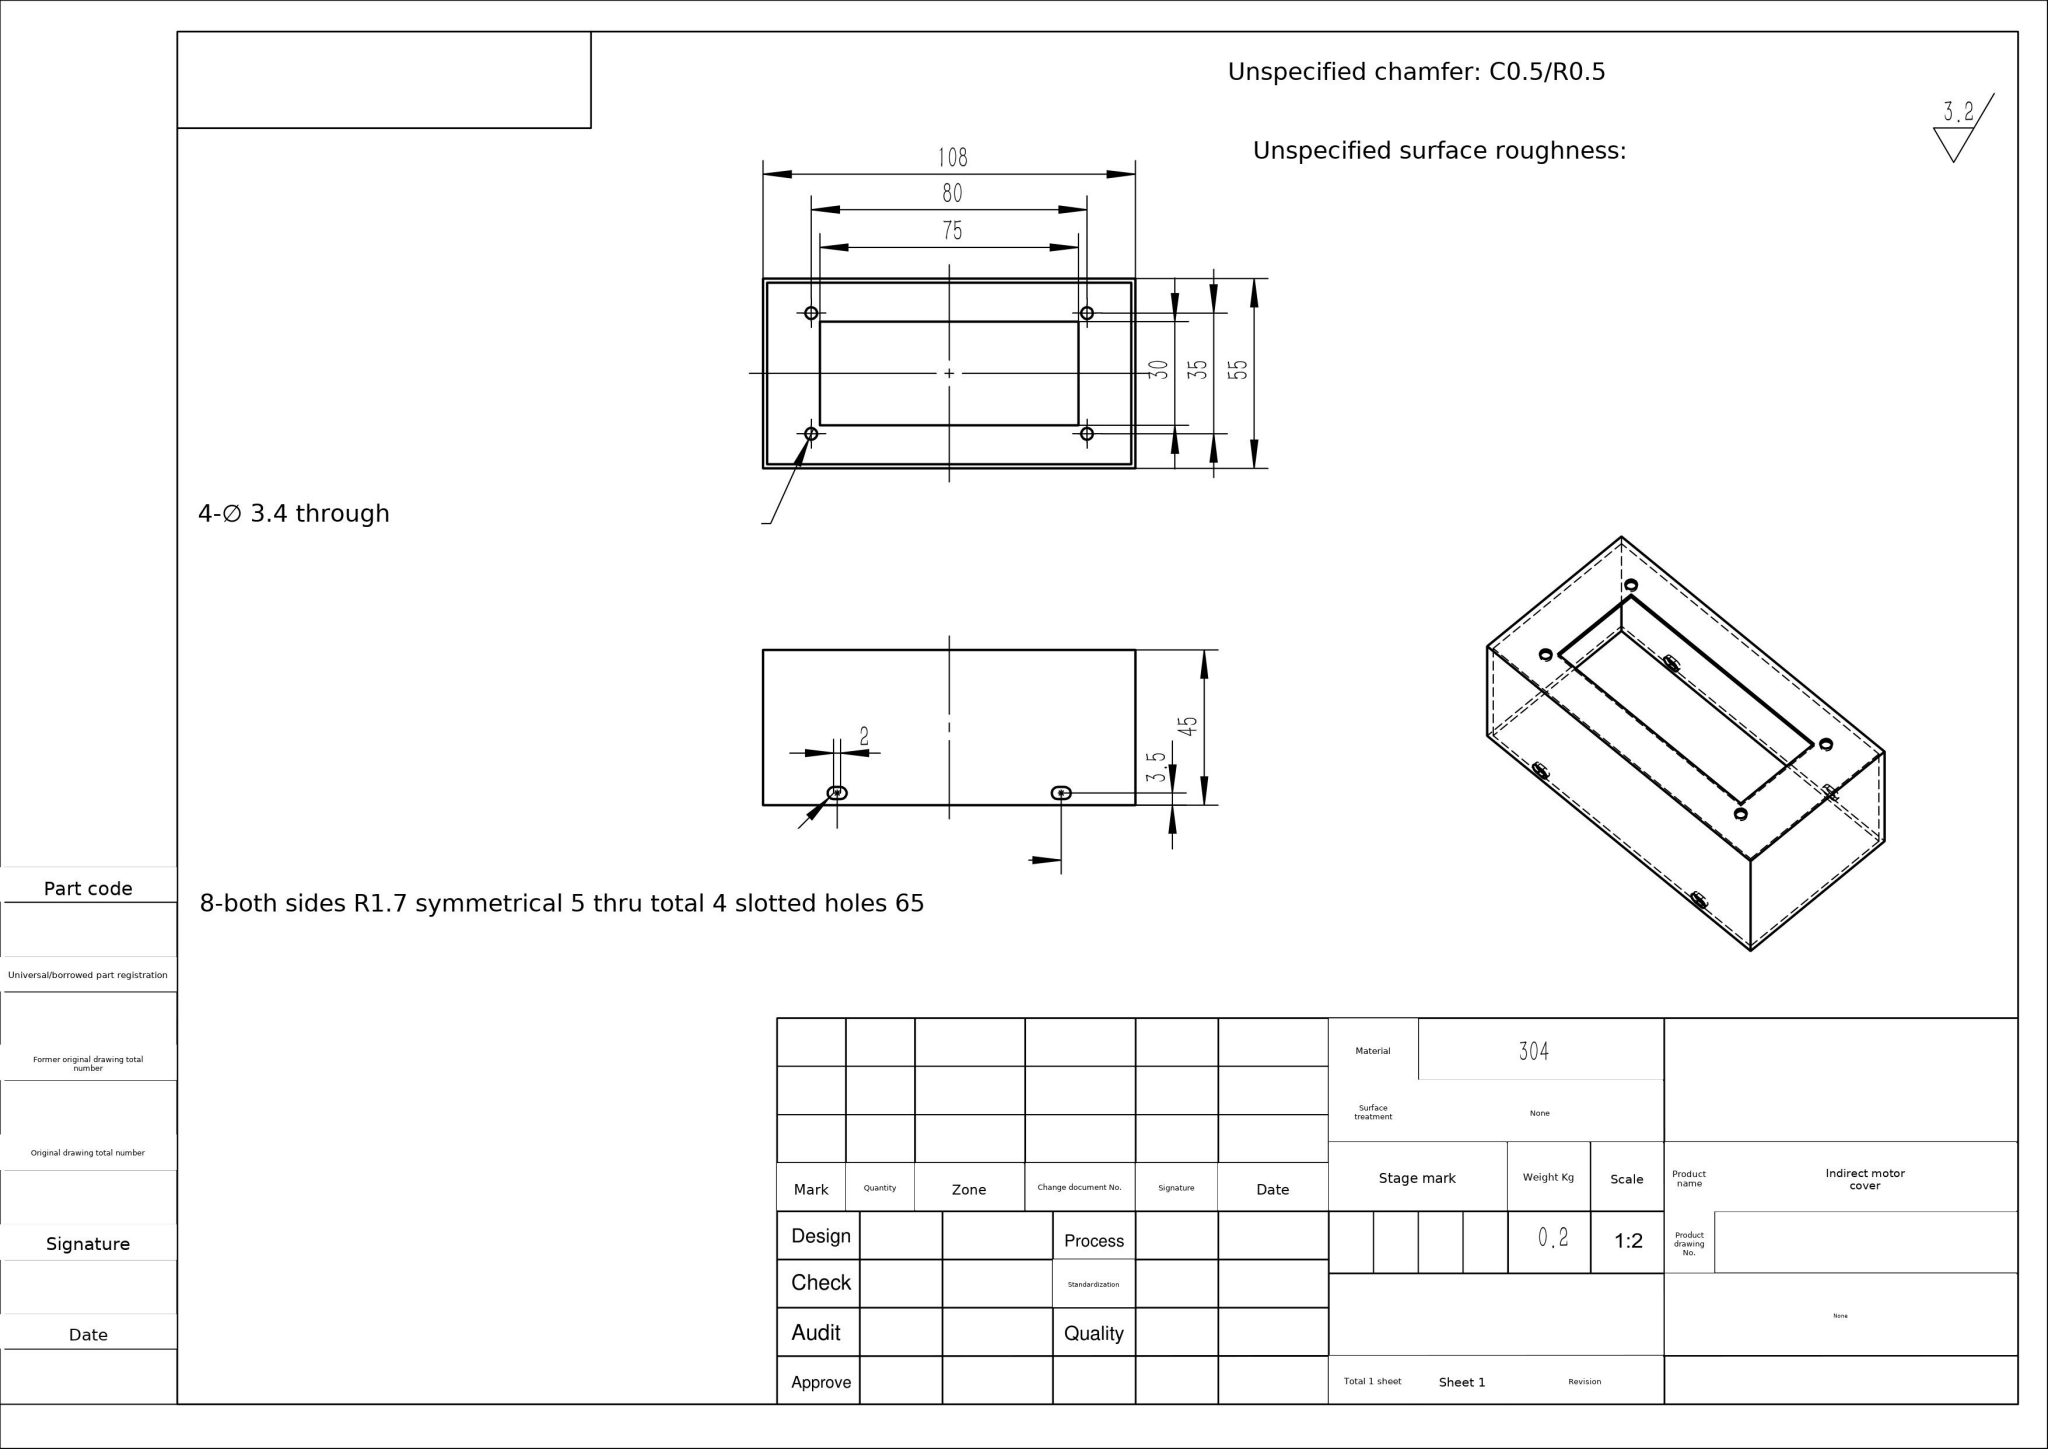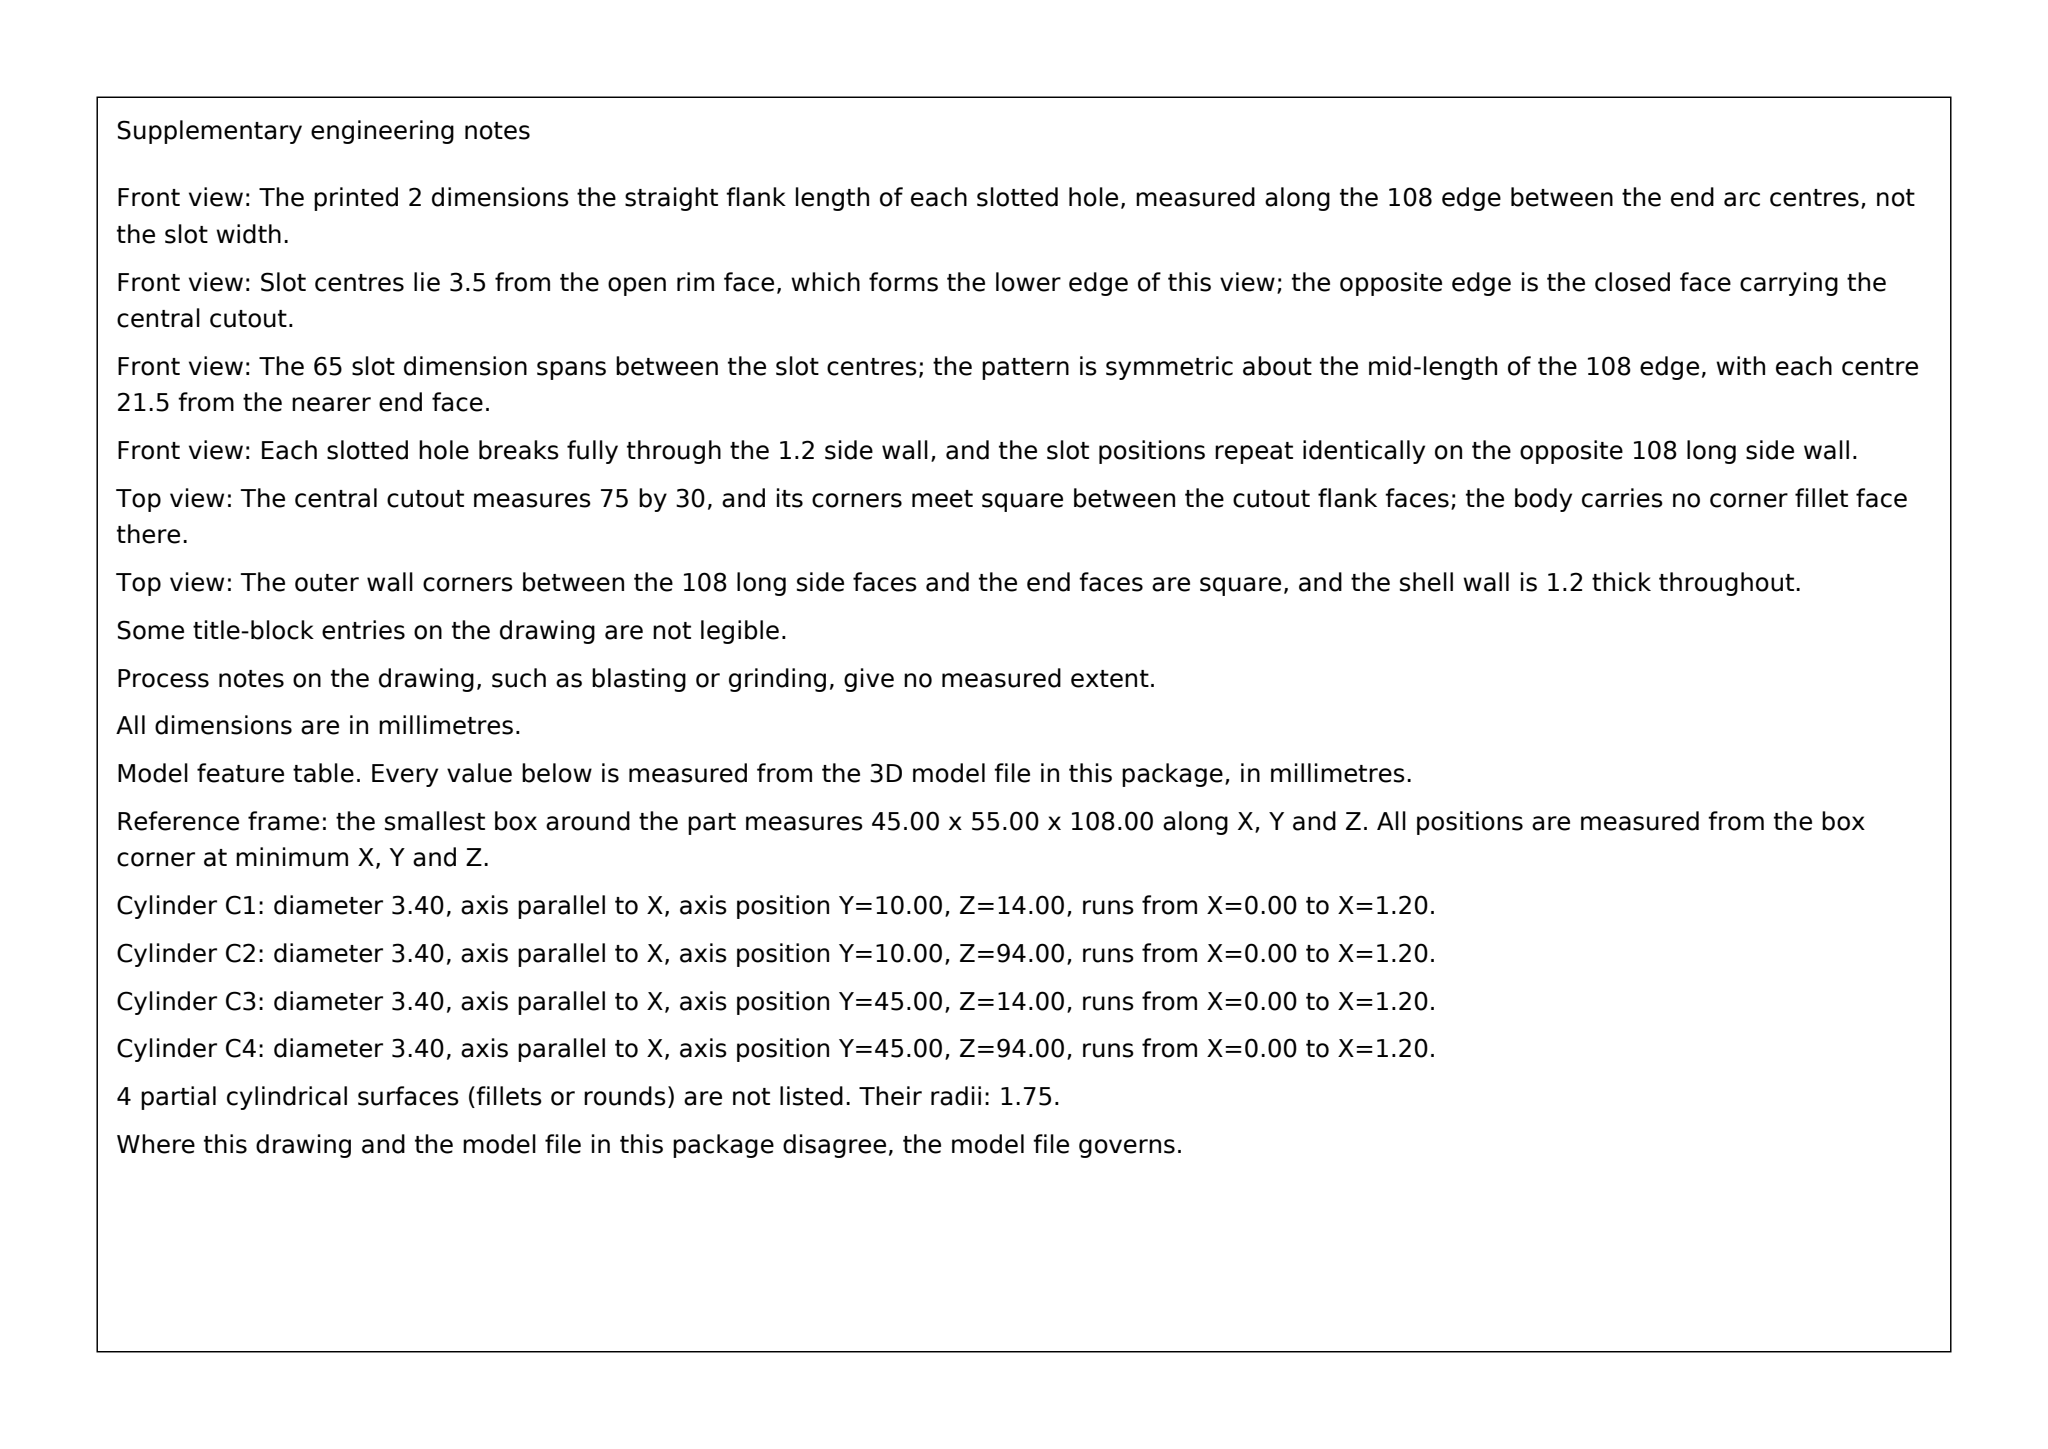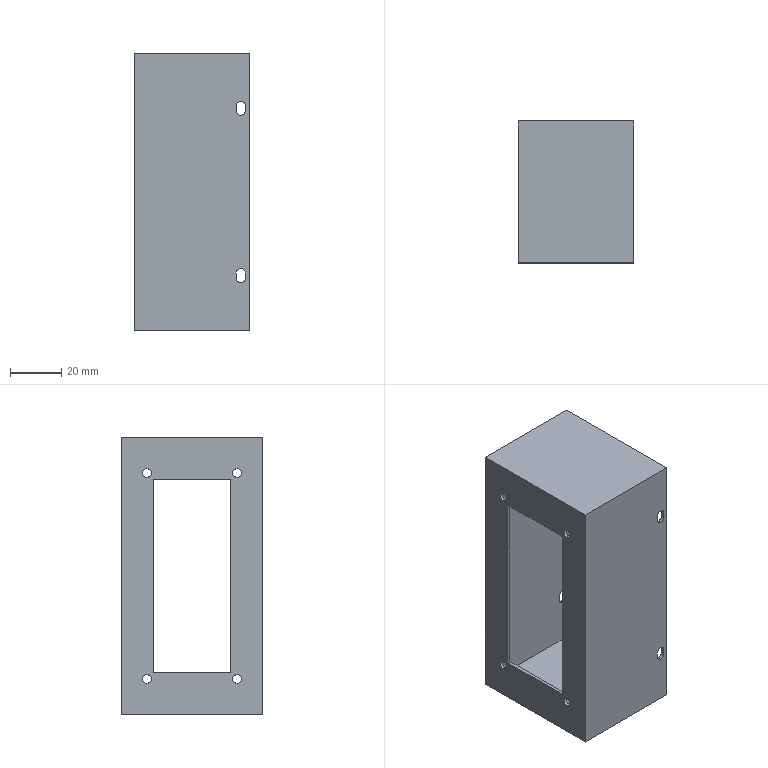Part | SolidWorks | mm | material 304 | 1 solid | 43 faces | box 45 x 55 x 108 mm | volume 21187 mm3 | plane 23 | cylinder 20 | commonest cylinder face diameters 3.5 x12 3.4 x8
Drawing notes:
8-SLOTS 3.5 W x 5.5 LG, R1.75 ENDS, 2 CTR-CTR, THRU BOTH SIDES | from the solid: Ø3.5 y-axis cyls at z=20.5 & 22.5 (and 85.5 & 87.5), len 1.2 thru walls y=0-1.2 / 53.8-55: slot width 3.5, ctr dist 2, overall 5.5, ends R1.75
4 SLOTTED HOLES: 65 C/C, SYM ABT CL OF 108 | from the solid: Slot arc centers z=21.5 (20.5/22.5) and z=86.5 (85.5/87.5): 86.5-21.5=65, sym about z=54 of 108 length
SHEET THK 1.2 TYP ALL WALLS | from the solid: Outer faces x=0,y=0,y=55,z=0,z=108 with inner faces at x=1.2, y=1.2, y=53.8, z=1.2, z=106.8
SLOT 3.5 WIDE X 5.5 LG, R1.75 ENDS, THRU 1.2 WALL | from the solid: Slot end arcs Ø3.5 (R1.75), centers 2 apart (20.5-22.5), y from 0 to 1.2 wall; overall 2+3.5=5.5
GARBLED LEADER '11 1.2' = WALL THK 1.2 | from the solid: Wall faces offset 1.2 from all outer faces; all holes/slots depth 0 to 1.2
SLOT CL 3.5 FROM OPEN EDGE, BOTH SIDE WALLS | from the solid: Slot arcs axis x=41.5; open rim face at x=45.0 -> 45.0-41.5=3.5
build123d program:
from build123d import *

# Parameters (mm, degrees)
SKETCH1_W                = 108
SKETCH1_H                = 55
BOSS_EXTRUDE1_DEPTH      = 45
SHELL1_T                 = -1.2
SKETCH3_W                = 75
SKETCH3_H                = 30
CUT_EXTRUDE2_DEPTH       = 10
M3_CLEARANCE_HOLE1_D     = 3.4
M3_CLEARANCE_HOLE1_DEPTH = 7.5
M3_CLEARANCE_HOLE1_TIP   = 1.021
CUT_EXTRUDE3_DEPTH       = 90.252


with BuildPart() as part:
    # Sketch1 → Boss-Extrude1 (new body)
    with BuildSketch(Plane(origin=(0, 0, 0), x_dir=(0, 0, -1), z_dir=(1, 0, 0))):
        Rectangle(SKETCH1_W, SKETCH1_H)
    extrude(amount=BOSS_EXTRUDE1_DEPTH)

    # Shell1
    shell1_openings = [part.faces().sort_by_distance(p)[0] for p in [
        (45, 0, 0),
    ]]
    offset(amount=SHELL1_T, openings=shell1_openings, kind=Kind.INTERSECTION)

    # Sketch3 → Cut-Extrude2 (cut)
    with BuildSketch(Plane.ZY):
        Rectangle(SKETCH3_W, SKETCH3_H)
    extrude(amount=-CUT_EXTRUDE2_DEPTH, mode=Mode.SUBTRACT)

    # M3 Clearance Hole1
    with Locations(Plane.ZY):
        with Locations((0, 0), (-40, 17.5), (40, -17.5), (40, 17.5), (-40, -17.5)):
            Hole(M3_CLEARANCE_HOLE1_D / 2, depth=M3_CLEARANCE_HOLE1_DEPTH)
            with Locations((0, 0, -(M3_CLEARANCE_HOLE1_DEPTH + M3_CLEARANCE_HOLE1_TIP / 2))):  # 118° drill point
                Cone(0, M3_CLEARANCE_HOLE1_D / 2, M3_CLEARANCE_HOLE1_TIP, mode=Mode.SUBTRACT)

    # Sketch7 → Cut-Extrude3 (cut, through all)
    with BuildSketch(Plane.XZ.offset(27.5)):
        with BuildLine():
            Line((39.75, 33.5), (39.75, 31.5))
            ThreePointArc((39.75, 31.5), (41.5, 29.75), (43.25, 31.5))
            Line((43.25, 31.5), (43.25, 33.5))
            ThreePointArc((43.25, 33.5), (41.5, 35.25), (39.75, 33.5))
        make_face()
        with BuildLine():
            Line((43.25, -33.5), (43.25, -31.5))
            ThreePointArc((43.25, -31.5), (41.5, -29.75), (39.75, -31.5))
            Line((39.75, -31.5), (39.75, -33.5))
            ThreePointArc((39.75, -33.5), (41.5, -35.25), (43.25, -33.5))
        make_face()
    extrude(amount=-CUT_EXTRUDE3_DEPTH, mode=Mode.SUBTRACT)


solid = part.part